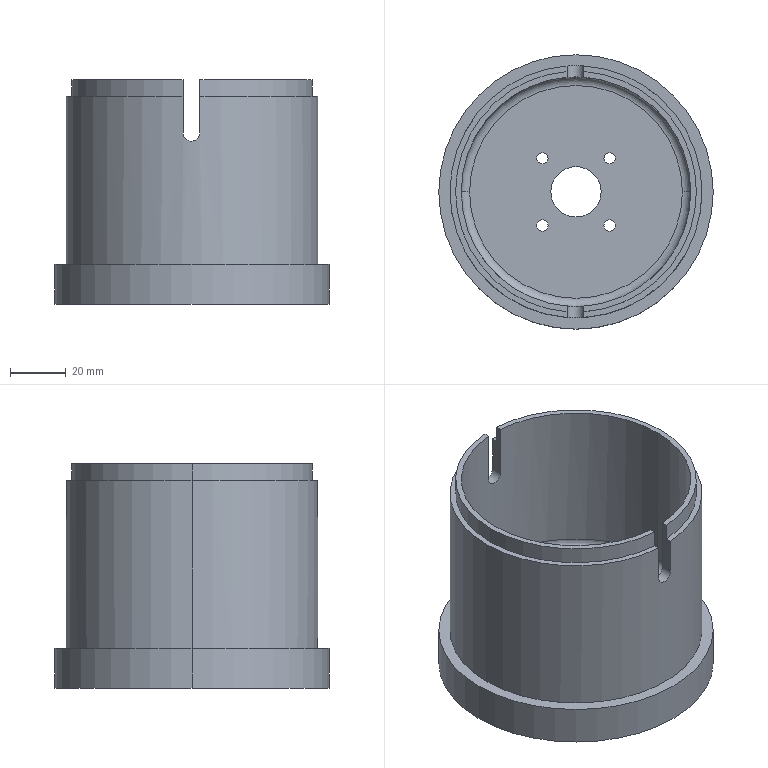Component | SolidWorks | g1-1 | 1 solid | 45 faces | volume 103166 mm3 | cylinder 27 | plane 14 | torus 4 | commonest cylinder face diameters 4 x8 82 x4 86 x3 94 x2 89.032 x2 98 x2 18 x2 90 x2